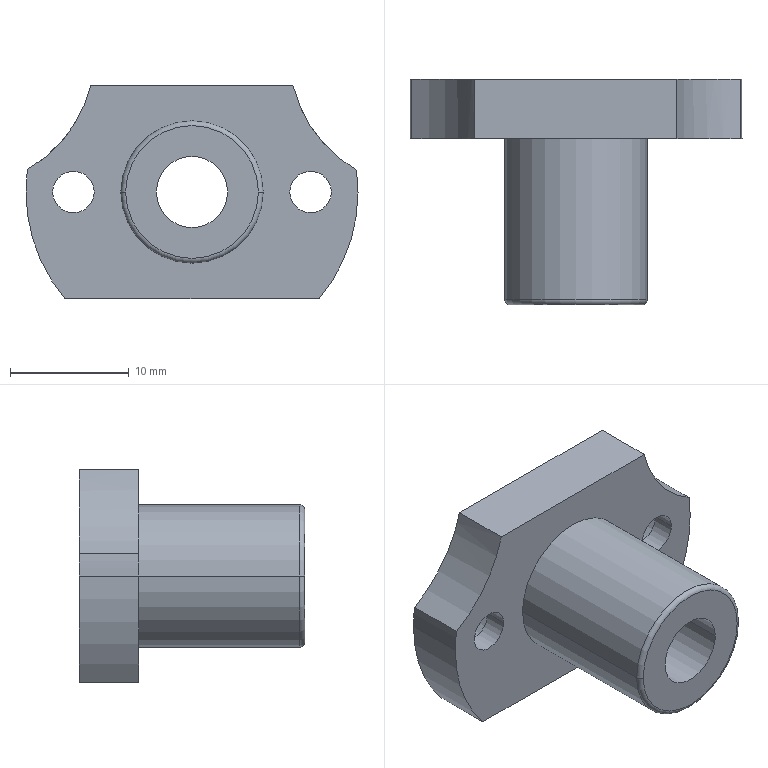Component | SolidWorks | LME21-d6-1 | 1 solid | 26 faces | box 28 x 19 x 18 mm | volume 3005 mm3 | cylinder 17 | plane 7 | torus 2 | commonest cylinder face diameters 6 x6 3.5 x4 28 x3 12 x2 22.6 x2
build123d program:
from build123d import *

# Parameters (mm, degrees)
BOSS_EXTRUDE1_START        = 5
SKETCH2_R                  = 6
BOSS_EXTRUDE1_DEPTH        = 5
FLANGENUTRELIEF_DEPTH      = 26.259
FLANGENUTRELIEF_DEPTH_BACK = 26.259
SKETCH1_R                  = 11.3


with BuildPart() as part:
    # Sketch1_2 → Revolve1 (revolve)
    with BuildSketch(Plane(origin=(0, 0, 0), x_dir=(1, 0, 0), z_dir=(0, 1, 0))):
        with BuildLine():
            Line((-5.6, -19), (-3, -19))
            Line((-3, -19), (-3, 0))
            Line((-3, 0), (-6, 0))
            Line((-6, 0), (-6, -18.6))
            ThreePointArc((-6, -18.6), (-5.883, -18.883), (-5.6, -19))
        make_face()
    revolve(axis=Axis((0, 0, 0), (0, 0, 1)))

    # Sketch2 → Boss-Extrude1 (add)
    with BuildSketch(Plane.XY.offset(BOSS_EXTRUDE1_START)):
        with BuildLine():
            Line((-10.724, -9), (10.724, -9))
            ThreePointArc((10.724, -9), (14, 0), (10.724, 9))
            Line((10.724, 9), (-10.724, 9))
            ThreePointArc((-10.724, 9), (-14, 0), (-10.724, -9))
        make_face()
        with Locations(Location((0, 0, 0), (0, 0, 180))):
            Circle(SKETCH2_R, mode=Mode.SUBTRACT)
    extrude(amount=-BOSS_EXTRUDE1_DEPTH)

    # Sketch3 → Cut-Revolve1 (revolve, cut)
    with BuildSketch(Plane(origin=(0, 0, 0), x_dir=(1, 0, 0), z_dir=(0, 1, 0))):
        Polygon((-10, -5), (-11.75, -5), (-11.75, -3.1), (-13, -3.1), (-13, 0), (-10, 0), align=None)
    revolve(axis=Axis((-10, 0, 0), (0, 0, 1)), mode=Mode.SUBTRACT)

    # Sketch4 → Cut-Revolve2 (revolve, cut)
    with BuildSketch(Plane(origin=(0, 0, 0), x_dir=(1, 0, 0), z_dir=(0, 1, 0))):
        Polygon((10, 0), (13, 0), (13, -3.1), (11.75, -3.1), (11.75, -5), (10, -5), align=None)
    revolve(axis=Axis((10, 0, 5), (0, 0, -1)), mode=Mode.SUBTRACT)

    # Sketch1 → FlangeNutRelief (cut, two sides: drawn at the far end of the back side and taken through both)
    with BuildSketch(Plane.XY.offset(-FLANGENUTRELIEF_DEPTH_BACK)):
        with Locations((19.5, 11.652)):
            Circle(SKETCH1_R)
        with Locations((-19.5, 11.704)):
            Circle(SKETCH1_R)
    extrude(amount=FLANGENUTRELIEF_DEPTH + FLANGENUTRELIEF_DEPTH_BACK, mode=Mode.SUBTRACT)


solid = part.part

# Placed as in the assembly
solid = solid.moved(Location((-57.536, 63.25, 217.788), (90, 0, 0)))
STEP:
#1=COLOUR_RGB('',0.7922,0.8196,0.9333);
#2=FILL_AREA_STYLE_COLOUR('',#1);
#3=FILL_AREA_STYLE('',(#2));
#4=SURFACE_STYLE_FILL_AREA(#3);
#5=SURFACE_SIDE_STYLE('',(#4));
#6=SURFACE_STYLE_USAGE(.BOTH.,#5);
#7=PRESENTATION_STYLE_ASSIGNMENT((#6));
#8=CARTESIAN_POINT('',(-1.94,2.368,8.574));
#9=VERTEX_POINT('',#8);
#10=CARTESIAN_POINT('',(-1.803,2.368,8.574));
#11=VERTEX_POINT('',#10);
#12=CARTESIAN_POINT('',(-1.872,2.368,8.574));
#13=DIRECTION('',(-0.,-1.,0.));
#14=DIRECTION('',(1.,-0.,0.));
#15=AXIS2_PLACEMENT_3D('',#12,#13,#14);
#16=CIRCLE('',#15,0.0689);
#17=EDGE_CURVE('',#9,#11,#16,.T.);
#18=ORIENTED_EDGE('',*,*,#17,.F.);
#19=CARTESIAN_POINT('',(-1.94,2.293,8.574));
#20=VERTEX_POINT('',#19);
#21=CARTESIAN_POINT('',(-1.94,2.293,8.574));
#22=DIRECTION('',(-0.,-1.,0.));
#23=VECTOR('',#22,39.37);
#24=LINE('',#21,#23);
#25=EDGE_CURVE('',#9,#20,#24,.T.);
#26=ORIENTED_EDGE('',*,*,#25,.T.);
#27=CARTESIAN_POINT('',(-1.803,2.293,8.574));
#28=VERTEX_POINT('',#27);
#29=CARTESIAN_POINT('',(-1.872,2.293,8.574));
#30=DIRECTION('',(-0.,-1.,0.));
#31=DIRECTION('',(1.,-0.,0.));
#32=AXIS2_PLACEMENT_3D('',#29,#30,#31);
#33=CIRCLE('',#32,0.0689);
#34=EDGE_CURVE('',#20,#28,#33,.T.);
#35=ORIENTED_EDGE('',*,*,#34,.T.);
#36=CARTESIAN_POINT('',(-1.803,2.293,8.574));
#37=DIRECTION('',(-0.,-1.,0.));
#38=VECTOR('',#37,39.37);
#39=LINE('',#36,#38);
#40=EDGE_CURVE('',#11,#28,#39,.T.);
#41=ORIENTED_EDGE('',*,*,#40,.F.);
#42=EDGE_LOOP('',(#18,#26,#35,#41));
#43=FACE_OUTER_BOUND('',#42,.T.);
#44=CARTESIAN_POINT('',(-1.872,2.293,8.574));
#45=DIRECTION('',(-0.,-1.,0.));
#46=DIRECTION('',(1.,-0.,0.));
#47=AXIS2_PLACEMENT_3D('',#44,#45,#46);
#48=CYLINDRICAL_SURFACE('',#47,0.0689);
#49=ADVANCED_FACE('',(#43),#48,.F.);
#50=CARTESIAN_POINT('',(-1.99,2.49,8.574));
#51=VERTEX_POINT('',#50);
#52=CARTESIAN_POINT('',(-1.753,2.49,8.574));
#53=VERTEX_POINT('',#52);
#54=CARTESIAN_POINT('',(-1.872,2.49,8.574));
#55=DIRECTION('',(-0.,-1.,0.));
#56=DIRECTION('',(1.,-0.,0.));
#57=AXIS2_PLACEMENT_3D('',#54,#55,#56);
#58=CIRCLE('',#57,0.1181);
#59=EDGE_CURVE('',#51,#53,#58,.T.);
#60=ORIENTED_EDGE('',*,*,#59,.F.);
#61=CARTESIAN_POINT('',(-1.99,2.368,8.574));
#62=VERTEX_POINT('',#61);
#63=CARTESIAN_POINT('',(-1.99,2.293,8.574));
#64=DIRECTION('',(-0.,-1.,0.));
#65=VECTOR('',#64,39.37);
#66=LINE('',#63,#65);
#67=EDGE_CURVE('',#51,#62,#66,.T.);
#68=ORIENTED_EDGE('',*,*,#67,.T.);
#69=CARTESIAN_POINT('',(-1.753,2.368,8.574));
#70=VERTEX_POINT('',#69);
#71=CARTESIAN_POINT('',(-1.872,2.368,8.574));
#72=DIRECTION('',(-0.,-1.,0.));
#73=DIRECTION('',(1.,-0.,0.));
#74=AXIS2_PLACEMENT_3D('',#71,#72,#73);
#75=CIRCLE('',#74,0.1181);
#76=EDGE_CURVE('',#62,#70,#75,.T.);
#77=ORIENTED_EDGE('',*,*,#76,.T.);
#78=CARTESIAN_POINT('',(-1.753,2.293,8.574));
#79=DIRECTION('',(-0.,-1.,0.));
#80=VECTOR('',#79,39.37);
#81=LINE('',#78,#80);
#82=EDGE_CURVE('',#53,#70,#81,.T.);
#83=ORIENTED_EDGE('',*,*,#82,.F.);
#84=EDGE_LOOP('',(#60,#68,#77,#83));
#85=FACE_OUTER_BOUND('',#84,.T.);
#86=CARTESIAN_POINT('',(-1.872,2.293,8.574));
#87=DIRECTION('',(-0.,-1.,0.));
#88=DIRECTION('',(1.,-0.,0.));
#89=AXIS2_PLACEMENT_3D('',#86,#87,#88);
#90=CYLINDRICAL_SURFACE('',#89,0.1181);
#91=ADVANCED_FACE('',(#85),#90,.F.);
#92=CARTESIAN_POINT('',(-2.541,2.368,8.574));
#93=VERTEX_POINT('',#92);
#94=CARTESIAN_POINT('',(-2.777,2.368,8.574));
#95=VERTEX_POINT('',#94);
#96=CARTESIAN_POINT('',(-2.659,2.368,8.574));
#97=DIRECTION('',(0.,1.,-0.));
#98=DIRECTION('',(-1.,0.,-0.));
#99=AXIS2_PLACEMENT_3D('',#96,#97,#98);
#100=CIRCLE('',#99,0.1181);
#101=EDGE_CURVE('',#93,#95,#100,.T.);
#102=ORIENTED_EDGE('',*,*,#101,.F.);
#103=CARTESIAN_POINT('',(-2.541,2.49,8.574));
#104=VERTEX_POINT('',#103);
#105=CARTESIAN_POINT('',(-2.541,2.49,8.574));
#106=DIRECTION('',(0.,1.,-0.));
#107=VECTOR('',#106,39.37);
#108=LINE('',#105,#107);
#109=EDGE_CURVE('',#93,#104,#108,.T.);
#110=ORIENTED_EDGE('',*,*,#109,.T.);
#111=CARTESIAN_POINT('',(-2.777,2.49,8.574));
#112=VERTEX_POINT('',#111);
#113=CARTESIAN_POINT('',(-2.659,2.49,8.574));
#114=DIRECTION('',(0.,1.,-0.));
#115=DIRECTION('',(-1.,0.,-0.));
#116=AXIS2_PLACEMENT_3D('',#113,#114,#115);
#117=CIRCLE('',#116,0.1181);
#118=EDGE_CURVE('',#104,#112,#117,.T.);
#119=ORIENTED_EDGE('',*,*,#118,.T.);
#120=CARTESIAN_POINT('',(-2.777,2.49,8.574));
#121=DIRECTION('',(0.,1.,-0.));
#122=VECTOR('',#121,39.37);
#123=LINE('',#120,#122);
#124=EDGE_CURVE('',#95,#112,#123,.T.);
#125=ORIENTED_EDGE('',*,*,#124,.F.);
#126=EDGE_LOOP('',(#102,#110,#119,#125));
#127=FACE_OUTER_BOUND('',#126,.T.);
#128=CARTESIAN_POINT('',(-2.659,2.49,8.574));
#129=DIRECTION('',(0.,1.,-0.));
#130=DIRECTION('',(-1.,0.,-0.));
#131=AXIS2_PLACEMENT_3D('',#128,#129,#130);
#132=CYLINDRICAL_SURFACE('',#131,0.1181);
#133=ADVANCED_FACE('',(#127),#132,.F.);
#134=CARTESIAN_POINT('',(-2.59,2.293,8.574));
#135=VERTEX_POINT('',#134);
#136=CARTESIAN_POINT('',(-2.728,2.293,8.574));
#137=VERTEX_POINT('',#136);
#138=CARTESIAN_POINT('',(-2.659,2.293,8.574));
#139=DIRECTION('',(0.,1.,-0.));
#140=DIRECTION('',(-1.,0.,0.));
#141=AXIS2_PLACEMENT_3D('',#138,#139,#140);
#142=CIRCLE('',#141,0.0689);
#143=EDGE_CURVE('',#135,#137,#142,.T.);
#144=ORIENTED_EDGE('',*,*,#143,.F.);
#145=CARTESIAN_POINT('',(-2.59,2.368,8.574));
#146=VERTEX_POINT('',#145);
#147=CARTESIAN_POINT('',(-2.59,2.49,8.574));
#148=DIRECTION('',(0.,1.,-0.));
#149=VECTOR('',#148,39.37);
#150=LINE('',#147,#149);
#151=EDGE_CURVE('',#135,#146,#150,.T.);
#152=ORIENTED_EDGE('',*,*,#151,.T.);
#153=CARTESIAN_POINT('',(-2.728,2.368,8.574));
#154=VERTEX_POINT('',#153);
#155=CARTESIAN_POINT('',(-2.659,2.368,8.574));
#156=DIRECTION('',(0.,1.,-0.));
#157=DIRECTION('',(-1.,0.,0.));
#158=AXIS2_PLACEMENT_3D('',#155,#156,#157);
#159=CIRCLE('',#158,0.0689);
#160=EDGE_CURVE('',#146,#154,#159,.T.);
#161=ORIENTED_EDGE('',*,*,#160,.T.);
#162=CARTESIAN_POINT('',(-2.728,2.49,8.574));
#163=DIRECTION('',(0.,1.,-0.));
#164=VECTOR('',#163,39.37);
#165=LINE('',#162,#164);
#166=EDGE_CURVE('',#137,#154,#165,.T.);
#167=ORIENTED_EDGE('',*,*,#166,.F.);
#168=EDGE_LOOP('',(#144,#152,#161,#167));
#169=FACE_OUTER_BOUND('',#168,.T.);
#170=CARTESIAN_POINT('',(-2.659,2.49,8.574));
#171=DIRECTION('',(0.,1.,-0.));
#172=DIRECTION('',(-1.,0.,0.));
#173=AXIS2_PLACEMENT_3D('',#170,#171,#172);
#174=CYLINDRICAL_SURFACE('',#173,0.0689);
#175=ADVANCED_FACE('',(#169),#174,.F.);
#176=CARTESIAN_POINT('',(-2.816,2.293,8.574));
#177=VERTEX_POINT('',#176);
#178=CARTESIAN_POINT('',(-2.687,2.293,8.22));
#179=VERTEX_POINT('',#178);
#180=CARTESIAN_POINT('',(-2.265,2.293,8.574));
#181=DIRECTION('',(-0.,-1.,0.));
#182=DIRECTION('',(1.,-0.,0.));
#183=AXIS2_PLACEMENT_3D('',#180,#181,#182);
#184=CIRCLE('',#183,0.5512);
#185=EDGE_CURVE('',#177,#179,#184,.T.);
#186=ORIENTED_EDGE('',*,*,#185,.F.);
#187=CARTESIAN_POINT('',(-2.816,2.49,8.574));
#188=VERTEX_POINT('',#187);
#189=CARTESIAN_POINT('',(-2.816,2.293,8.574));
#190=DIRECTION('',(0.,1.,-0.));
#191=VECTOR('',#190,39.37);
#192=LINE('',#189,#191);
#193=EDGE_CURVE('',#177,#188,#192,.T.);
#194=ORIENTED_EDGE('',*,*,#193,.T.);
#195=CARTESIAN_POINT('',(-2.687,2.49,8.22));
#196=VERTEX_POINT('',#195);
#197=CARTESIAN_POINT('',(-2.265,2.49,8.574));
#198=DIRECTION('',(-0.,-1.,0.));
#199=DIRECTION('',(1.,-0.,0.));
#200=AXIS2_PLACEMENT_3D('',#197,#198,#199);
#201=CIRCLE('',#200,0.5512);
#202=EDGE_CURVE('',#188,#196,#201,.T.);
#203=ORIENTED_EDGE('',*,*,#202,.T.);
#204=CARTESIAN_POINT('',(-2.687,2.293,8.22));
#205=DIRECTION('',(0.,1.,-0.));
#206=VECTOR('',#205,39.37);
#207=LINE('',#204,#206);
#208=EDGE_CURVE('',#179,#196,#207,.T.);
#209=ORIENTED_EDGE('',*,*,#208,.F.);
#210=EDGE_LOOP('',(#186,#194,#203,#209));
#211=FACE_OUTER_BOUND('',#210,.T.);
#212=CARTESIAN_POINT('',(-2.265,2.293,8.574));
#213=DIRECTION('',(0.,1.,-0.));
#214=DIRECTION('',(-1.,0.,-0.));
#215=AXIS2_PLACEMENT_3D('',#212,#213,#214);
#216=CYLINDRICAL_SURFACE('',#215,0.5512);
#217=ADVANCED_FACE('',(#211),#216,.T.);
#218=CARTESIAN_POINT('',(-2.501,1.758,8.574));
#219=VERTEX_POINT('',#218);
#220=CARTESIAN_POINT('',(-2.029,1.758,8.574));
#221=VERTEX_POINT('',#220);
#222=CARTESIAN_POINT('',(-2.265,1.758,8.574));
#223=DIRECTION('',(0.,1.,-0.));
#224=DIRECTION('',(-1.,0.,-0.));
#225=AXIS2_PLACEMENT_3D('',#222,#223,#224);
#226=CIRCLE('',#225,0.2362);
#227=EDGE_CURVE('',#219,#221,#226,.T.);
#228=ORIENTED_EDGE('',*,*,#227,.T.);
#229=CARTESIAN_POINT('',(-2.029,2.293,8.574));
#230=VERTEX_POINT('',#229);
#231=CARTESIAN_POINT('',(-2.029,2.49,8.574));
#232=DIRECTION('',(0.,1.,-0.));
#233=VECTOR('',#232,39.37);
#234=LINE('',#231,#233);
#235=EDGE_CURVE('',#221,#230,#234,.T.);
#236=ORIENTED_EDGE('',*,*,#235,.T.);
#237=CARTESIAN_POINT('',(-2.501,2.293,8.574));
#238=VERTEX_POINT('',#237);
#239=CARTESIAN_POINT('',(-2.265,2.293,8.574));
#240=DIRECTION('',(0.,1.,-0.));
#241=DIRECTION('',(1.,-0.,0.));
#242=AXIS2_PLACEMENT_3D('',#239,#240,#241);
#243=CIRCLE('',#242,0.2362);
#244=EDGE_CURVE('',#238,#230,#243,.T.);
#245=ORIENTED_EDGE('',*,*,#244,.F.);
#246=CARTESIAN_POINT('',(-2.501,2.49,8.574));
#247=DIRECTION('',(0.,1.,-0.));
#248=VECTOR('',#247,39.37);
#249=LINE('',#246,#248);
#250=EDGE_CURVE('',#219,#238,#249,.T.);
#251=ORIENTED_EDGE('',*,*,#250,.F.);
#252=EDGE_LOOP('',(#228,#236,#245,#251));
#253=FACE_OUTER_BOUND('',#252,.T.);
#254=CARTESIAN_POINT('',(-2.265,2.49,8.574));
#255=DIRECTION('',(0.,1.,-0.));
#256=DIRECTION('',(-1.,0.,-0.));
#257=AXIS2_PLACEMENT_3D('',#254,#255,#256);
#258=CYLINDRICAL_SURFACE('',#257,0.2362);
#259=ADVANCED_FACE('',(#253),#258,.T.);
#260=CARTESIAN_POINT('',(-2.147,1.742,8.574));
#261=VERTEX_POINT('',#260);
#262=CARTESIAN_POINT('',(-2.383,1.742,8.574));
#263=VERTEX_POINT('',#262);
#264=CARTESIAN_POINT('',(-2.265,1.742,8.574));
#265=DIRECTION('',(0.,1.,-0.));
#266=DIRECTION('',(-1.,0.,-0.));
#267=AXIS2_PLACEMENT_3D('',#264,#265,#266);
#268=CIRCLE('',#267,0.1181);
#269=EDGE_CURVE('',#261,#263,#268,.T.);
#270=ORIENTED_EDGE('',*,*,#269,.F.);
#271=CARTESIAN_POINT('',(-2.147,2.49,8.574));
#272=VERTEX_POINT('',#271);
#273=CARTESIAN_POINT('',(-2.147,2.49,8.574));
#274=DIRECTION('',(0.,1.,-0.));
#275=VECTOR('',#274,39.37);
#276=LINE('',#273,#275);
#277=EDGE_CURVE('',#261,#272,#276,.T.);
#278=ORIENTED_EDGE('',*,*,#277,.T.);
#279=CARTESIAN_POINT('',(-2.383,2.49,8.574));
#280=VERTEX_POINT('',#279);
#281=CARTESIAN_POINT('',(-2.265,2.49,8.574));
#282=DIRECTION('',(0.,1.,-0.));
#283=DIRECTION('',(-1.,0.,-0.));
#284=AXIS2_PLACEMENT_3D('',#281,#282,#283);
#285=CIRCLE('',#284,0.1181);
#286=EDGE_CURVE('',#272,#280,#285,.T.);
#287=ORIENTED_EDGE('',*,*,#286,.T.);
#288=CARTESIAN_POINT('',(-2.383,2.49,8.574));
#289=DIRECTION('',(0.,1.,-0.));
#290=VECTOR('',#289,39.37);
#291=LINE('',#288,#290);
#292=EDGE_CURVE('',#263,#280,#291,.T.);
#293=ORIENTED_EDGE('',*,*,#292,.F.);
#294=EDGE_LOOP('',(#270,#278,#287,#293));
#295=FACE_OUTER_BOUND('',#294,.T.);
#296=CARTESIAN_POINT('',(-2.265,2.49,8.574));
#297=DIRECTION('',(0.,1.,-0.));
#298=DIRECTION('',(-1.,0.,-0.));
#299=AXIS2_PLACEMENT_3D('',#296,#297,#298);
#300=CYLINDRICAL_SURFACE('',#299,0.1181);
#301=ADVANCED_FACE('',(#295),#300,.F.);
#302=CARTESIAN_POINT('',(-2.486,1.742,8.574));
#303=VERTEX_POINT('',#302);
#304=CARTESIAN_POINT('',(-2.045,1.742,8.574));
#305=VERTEX_POINT('',#304);
#306=CARTESIAN_POINT('',(-2.265,1.742,8.574));
#307=DIRECTION('',(0.,1.,-0.));
#308=DIRECTION('',(-1.,0.,-0.));
#309=AXIS2_PLACEMENT_3D('',#306,#307,#308);
#310=CIRCLE('',#309,0.2205);
#311=EDGE_CURVE('',#303,#305,#310,.T.);
#312=ORIENTED_EDGE('',*,*,#311,.T.);
#313=CARTESIAN_POINT('',(-2.045,1.758,8.574));
#314=DIRECTION('',(-0.,0.,1.));
#315=DIRECTION('',(1.,0.,0.));
#316=AXIS2_PLACEMENT_3D('',#313,#314,#315);
#317=CIRCLE('',#316,0.01575);
#318=EDGE_CURVE('',#305,#221,#317,.T.);
#319=ORIENTED_EDGE('',*,*,#318,.T.);
#320=ORIENTED_EDGE('',*,*,#227,.F.);
#321=CARTESIAN_POINT('',(-2.486,1.758,8.574));
#322=DIRECTION('',(0.,-0.,-1.));
#323=DIRECTION('',(-1.,0.,0.));
#324=AXIS2_PLACEMENT_3D('',#321,#322,#323);
#325=CIRCLE('',#324,0.01575);
#326=EDGE_CURVE('',#303,#219,#325,.T.);
#327=ORIENTED_EDGE('',*,*,#326,.F.);
#328=EDGE_LOOP('',(#312,#319,#320,#327));
#329=FACE_OUTER_BOUND('',#328,.T.);
#330=CARTESIAN_POINT('',(-2.265,1.758,8.574));
#331=DIRECTION('',(0.,1.,-0.));
#332=DIRECTION('',(-1.,0.,-0.));
#333=AXIS2_PLACEMENT_3D('',#330,#331,#332);
#334=TOROIDAL_SURFACE('',#333,0.2205,0.01575);
#335=ADVANCED_FACE('',(#329),#334,.T.);
#336=CARTESIAN_POINT('',(-1.872,2.49,8.574));
#337=DIRECTION('',(-0.,-1.,0.));
#338=DIRECTION('',(1.,-0.,0.));
#339=AXIS2_PLACEMENT_3D('',#336,#337,#338);
#340=CIRCLE('',#339,0.1181);
#341=EDGE_CURVE('',#53,#51,#340,.T.);
#342=ORIENTED_EDGE('',*,*,#341,.T.);
#343=ORIENTED_EDGE('',*,*,#59,.T.);
#344=EDGE_LOOP('',(#342,#343));
#345=FACE_BOUND('',#344,.T.);
#346=CARTESIAN_POINT('',(-2.659,2.49,8.574));
#347=DIRECTION('',(0.,1.,-0.));
#348=DIRECTION('',(-1.,0.,-0.));
#349=AXIS2_PLACEMENT_3D('',#346,#347,#348);
#350=CIRCLE('',#349,0.1181);
#351=EDGE_CURVE('',#112,#104,#350,.T.);
#352=ORIENTED_EDGE('',*,*,#351,.F.);
#353=ORIENTED_EDGE('',*,*,#118,.F.);
#354=EDGE_LOOP('',(#352,#353));
#355=FACE_BOUND('',#354,.T.);
#356=CARTESIAN_POINT('',(-2.265,2.49,8.574));
#357=DIRECTION('',(0.,1.,-0.));
#358=DIRECTION('',(-1.,0.,-0.));
#359=AXIS2_PLACEMENT_3D('',#356,#357,#358);
#360=CIRCLE('',#359,0.1181);
#361=EDGE_CURVE('',#280,#272,#360,.T.);
#362=ORIENTED_EDGE('',*,*,#361,.F.);
#363=ORIENTED_EDGE('',*,*,#286,.F.);
#364=EDGE_LOOP('',(#362,#363));
#365=FACE_BOUND('',#364,.T.);
#366=CARTESIAN_POINT('',(-1.93,2.49,8.929));
#367=VERTEX_POINT('',#366);
#368=CARTESIAN_POINT('',(-2.601,2.49,8.929));
#369=VERTEX_POINT('',#368);
#370=CARTESIAN_POINT('',(-1.843,2.49,8.929));
#371=DIRECTION('',(-1.,0.,-0.));
#372=VECTOR('',#371,39.37);
#373=LINE('',#370,#372);
#374=EDGE_CURVE('',#367,#369,#373,.T.);
#375=ORIENTED_EDGE('',*,*,#374,.F.);
#376=CARTESIAN_POINT('',(-1.719,2.49,8.647));
#377=VERTEX_POINT('',#376);
#378=CARTESIAN_POINT('',(-1.93,2.49,8.929));
#379=CARTESIAN_POINT('',(-1.926,2.49,8.914));
#380=CARTESIAN_POINT('',(-1.922,2.49,8.9));
#381=CARTESIAN_POINT('',(-1.912,2.49,8.871));
#382=CARTESIAN_POINT('',(-1.906,2.49,8.857));
#383=CARTESIAN_POINT('',(-1.887,2.49,8.816));
#384=CARTESIAN_POINT('',(-1.864,2.49,8.777));
#385=CARTESIAN_POINT('',(-1.835,2.49,8.743));
#386=CARTESIAN_POINT('',(-1.814,2.49,8.72));
#387=CARTESIAN_POINT('',(-1.803,2.49,8.71));
#388=CARTESIAN_POINT('',(-1.769,2.49,8.679));
#389=CARTESIAN_POINT('',(-1.745,2.49,8.662));
#390=CARTESIAN_POINT('',(-1.719,2.49,8.647));
#391=B_SPLINE_CURVE_WITH_KNOTS('',3,(#378,#379,#380,#381,#382,#383,#384,#385,#386,#387,#388,#389,#390),.UNSPECIFIED.,.F.,.F.,(4,2,2,1,2,2,4),(0.5377,0.5539,0.5701,0.6025,0.6186,0.6348,0.6672),.UNSPECIFIED.);
#392=EDGE_CURVE('',#367,#377,#391,.T.);
#393=ORIENTED_EDGE('',*,*,#392,.T.);
#394=CARTESIAN_POINT('',(-1.843,2.49,8.22));
#395=VERTEX_POINT('',#394);
#396=CARTESIAN_POINT('',(-2.265,2.49,8.574));
#397=DIRECTION('',(-0.,-1.,0.));
#398=DIRECTION('',(1.,-0.,0.));
#399=AXIS2_PLACEMENT_3D('',#396,#397,#398);
#400=CIRCLE('',#399,0.5512);
#401=EDGE_CURVE('',#395,#377,#400,.T.);
#402=ORIENTED_EDGE('',*,*,#401,.F.);
#403=CARTESIAN_POINT('',(-2.687,2.49,8.22));
#404=DIRECTION('',(1.,-0.,0.));
#405=VECTOR('',#404,39.37);
#406=LINE('',#403,#405);
#407=EDGE_CURVE('',#196,#395,#406,.T.);
#408=ORIENTED_EDGE('',*,*,#407,.F.);
#409=ORIENTED_EDGE('',*,*,#202,.F.);
#410=CARTESIAN_POINT('',(-2.811,2.49,8.649));
#411=VERTEX_POINT('',#410);
#412=CARTESIAN_POINT('',(-2.265,2.49,8.574));
#413=DIRECTION('',(-0.,-1.,0.));
#414=DIRECTION('',(1.,-0.,0.));
#415=AXIS2_PLACEMENT_3D('',#412,#413,#414);
#416=CIRCLE('',#415,0.5512);
#417=EDGE_CURVE('',#411,#188,#416,.T.);
#418=ORIENTED_EDGE('',*,*,#417,.F.);
#419=CARTESIAN_POINT('',(-2.811,2.49,8.649));
#420=CARTESIAN_POINT('',(-2.785,2.49,8.664));
#421=CARTESIAN_POINT('',(-2.761,2.49,8.682));
#422=CARTESIAN_POINT('',(-2.727,2.49,8.711));
#423=CARTESIAN_POINT('',(-2.717,2.49,8.722));
#424=CARTESIAN_POINT('',(-2.696,2.49,8.744));
#425=CARTESIAN_POINT('',(-2.667,2.49,8.779));
#426=CARTESIAN_POINT('',(-2.644,2.49,8.817));
#427=CARTESIAN_POINT('',(-2.625,2.49,8.858));
#428=CARTESIAN_POINT('',(-2.619,2.49,8.872));
#429=CARTESIAN_POINT('',(-2.609,2.49,8.9));
#430=CARTESIAN_POINT('',(-2.604,2.49,8.914));
#431=CARTESIAN_POINT('',(-2.601,2.49,8.929));
#432=B_SPLINE_CURVE_WITH_KNOTS('',3,(#419,#420,#421,#422,#423,#424,#425,#426,#427,#428,#429,#430,#431),.UNSPECIFIED.,.F.,.F.,(4,2,2,1,2,2,4),(0.8329,0.8651,0.8812,0.8972,0.9294,0.9454,0.9615),.UNSPECIFIED.);
#433=EDGE_CURVE('',#411,#369,#432,.T.);
#434=ORIENTED_EDGE('',*,*,#433,.T.);
#435=EDGE_LOOP('',(#375,#393,#402,#408,#409,#418,#434));
#436=FACE_OUTER_BOUND('',#435,.T.);
#437=CARTESIAN_POINT('',(-2.383,2.49,8.574));
#438=DIRECTION('',(0.,1.,-0.));
#439=DIRECTION('',(-1.,0.,-0.));
#440=AXIS2_PLACEMENT_3D('',#437,#438,#439);
#441=PLANE('',#440);
#442=ADVANCED_FACE('',(#345,#355,#365,#436),#441,.T.);
#443=ORIENTED_EDGE('',*,*,#318,.F.);
#444=CARTESIAN_POINT('',(-2.265,1.742,8.574));
#445=DIRECTION('',(0.,1.,-0.));
#446=DIRECTION('',(-1.,0.,-0.));
#447=AXIS2_PLACEMENT_3D('',#444,#445,#446);
#448=CIRCLE('',#447,0.2205);
#449=EDGE_CURVE('',#305,#303,#448,.T.);
#450=ORIENTED_EDGE('',*,*,#449,.T.);
#451=ORIENTED_EDGE('',*,*,#326,.T.);
#452=CARTESIAN_POINT('',(-2.265,1.758,8.574));
#453=DIRECTION('',(0.,1.,-0.));
#454=DIRECTION('',(-1.,0.,-0.));
#455=AXIS2_PLACEMENT_3D('',#452,#453,#454);
#456=CIRCLE('',#455,0.2362);
#457=EDGE_CURVE('',#221,#219,#456,.T.);
#458=ORIENTED_EDGE('',*,*,#457,.F.);
#459=EDGE_LOOP('',(#443,#450,#451,#458));
#460=FACE_OUTER_BOUND('',#459,.T.);
#461=CARTESIAN_POINT('',(-2.265,1.758,8.574));
#462=DIRECTION('',(0.,1.,-0.));
#463=DIRECTION('',(-1.,0.,-0.));
#464=AXIS2_PLACEMENT_3D('',#461,#462,#463);
#465=TOROIDAL_SURFACE('',#464,0.2205,0.01575);
#466=ADVANCED_FACE('',(#460),#465,.T.);
#467=CARTESIAN_POINT('',(-2.265,1.742,8.574));
#468=DIRECTION('',(0.,1.,-0.));
#469=DIRECTION('',(-1.,0.,-0.));
#470=AXIS2_PLACEMENT_3D('',#467,#468,#469);
#471=CIRCLE('',#470,0.1181);
#472=EDGE_CURVE('',#263,#261,#471,.T.);
#473=ORIENTED_EDGE('',*,*,#472,.T.);
#474=ORIENTED_EDGE('',*,*,#269,.T.);
#475=EDGE_LOOP('',(#473,#474));
#476=FACE_BOUND('',#475,.T.);
#477=ORIENTED_EDGE('',*,*,#311,.F.);
#478=ORIENTED_EDGE('',*,*,#449,.F.);
#479=EDGE_LOOP('',(#477,#478));
#480=FACE_OUTER_BOUND('',#479,.T.);
#481=CARTESIAN_POINT('',(-2.486,1.742,8.574));
#482=DIRECTION('',(-0.,-1.,0.));
#483=DIRECTION('',(1.,-0.,0.));
#484=AXIS2_PLACEMENT_3D('',#481,#482,#483);
#485=PLANE('',#484);
#486=ADVANCED_FACE('',(#476,#480),#485,.T.);
#487=ORIENTED_EDGE('',*,*,#277,.F.);
#488=ORIENTED_EDGE('',*,*,#472,.F.);
#489=ORIENTED_EDGE('',*,*,#292,.T.);
#490=ORIENTED_EDGE('',*,*,#361,.T.);
#491=EDGE_LOOP('',(#487,#488,#489,#490));
#492=FACE_OUTER_BOUND('',#491,.T.);
#493=CARTESIAN_POINT('',(-2.265,2.49,8.574));
#494=DIRECTION('',(0.,1.,-0.));
#495=DIRECTION('',(-1.,0.,-0.));
#496=AXIS2_PLACEMENT_3D('',#493,#494,#495);
#497=CYLINDRICAL_SURFACE('',#496,0.1181);
#498=ADVANCED_FACE('',(#492),#497,.F.);
#499=ORIENTED_EDGE('',*,*,#235,.F.);
#500=ORIENTED_EDGE('',*,*,#457,.T.);
#501=ORIENTED_EDGE('',*,*,#250,.T.);
#502=CARTESIAN_POINT('',(-2.265,2.293,8.574));
#503=DIRECTION('',(0.,1.,-0.));
#504=DIRECTION('',(1.,-0.,0.));
#505=AXIS2_PLACEMENT_3D('',#502,#503,#504);
#506=CIRCLE('',#505,0.2362);
#507=EDGE_CURVE('',#230,#238,#506,.T.);
#508=ORIENTED_EDGE('',*,*,#507,.F.);
#509=EDGE_LOOP('',(#499,#500,#501,#508));
#510=FACE_OUTER_BOUND('',#509,.T.);
#511=CARTESIAN_POINT('',(-2.265,2.49,8.574));
#512=DIRECTION('',(0.,1.,-0.));
#513=DIRECTION('',(-1.,0.,-0.));
#514=AXIS2_PLACEMENT_3D('',#511,#512,#513);
#515=CYLINDRICAL_SURFACE('',#514,0.2362);
#516=ADVANCED_FACE('',(#510),#515,.T.);
#517=CARTESIAN_POINT('',(-1.93,2.293,8.929));
#518=VERTEX_POINT('',#517);
#519=CARTESIAN_POINT('',(-1.719,2.293,8.647));
#520=VERTEX_POINT('',#519);
#521=CARTESIAN_POINT('',(-1.497,2.293,9.033));
#522=DIRECTION('',(-0.,-1.,0.));
#523=DIRECTION('',(1.,-0.,0.));
#524=AXIS2_PLACEMENT_3D('',#521,#522,#523);
#525=CIRCLE('',#524,0.4449);
#526=EDGE_CURVE('',#518,#520,#525,.T.);
#527=ORIENTED_EDGE('',*,*,#526,.F.);
#528=CARTESIAN_POINT('',(-2.601,2.293,8.929));
#529=VERTEX_POINT('',#528);
#530=CARTESIAN_POINT('',(-1.843,2.293,8.929));
#531=DIRECTION('',(-1.,0.,-0.));
#532=VECTOR('',#531,39.37);
#533=LINE('',#530,#532);
#534=EDGE_CURVE('',#518,#529,#533,.T.);
#535=ORIENTED_EDGE('',*,*,#534,.T.);
#536=CARTESIAN_POINT('',(-2.811,2.293,8.649));
#537=VERTEX_POINT('',#536);
#538=CARTESIAN_POINT('',(-3.033,2.293,9.035));
#539=DIRECTION('',(-0.,-1.,0.));
#540=DIRECTION('',(1.,-0.,0.));
#541=AXIS2_PLACEMENT_3D('',#538,#539,#540);
#542=CIRCLE('',#541,0.4449);
#543=EDGE_CURVE('',#537,#529,#542,.T.);
#544=ORIENTED_EDGE('',*,*,#543,.F.);
#545=CARTESIAN_POINT('',(-2.265,2.293,8.574));
#546=DIRECTION('',(-0.,-1.,0.));
#547=DIRECTION('',(1.,-0.,0.));
#548=AXIS2_PLACEMENT_3D('',#545,#546,#547);
#549=CIRCLE('',#548,0.5512);
#550=EDGE_CURVE('',#537,#177,#549,.T.);
#551=ORIENTED_EDGE('',*,*,#550,.T.);
#552=ORIENTED_EDGE('',*,*,#185,.T.);
#553=CARTESIAN_POINT('',(-1.843,2.293,8.22));
#554=VERTEX_POINT('',#553);
#555=CARTESIAN_POINT('',(-2.687,2.293,8.22));
#556=DIRECTION('',(1.,-0.,0.));
#557=VECTOR('',#556,39.37);
#558=LINE('',#555,#557);
#559=EDGE_CURVE('',#179,#554,#558,.T.);
#560=ORIENTED_EDGE('',*,*,#559,.T.);
#561=CARTESIAN_POINT('',(-2.265,2.293,8.574));
#562=DIRECTION('',(-0.,-1.,0.));
#563=DIRECTION('',(1.,-0.,0.));
#564=AXIS2_PLACEMENT_3D('',#561,#562,#563);
#565=CIRCLE('',#564,0.5512);
#566=EDGE_CURVE('',#554,#520,#565,.T.);
#567=ORIENTED_EDGE('',*,*,#566,.T.);
#568=EDGE_LOOP('',(#527,#535,#544,#551,#552,#560,#567));
#569=FACE_OUTER_BOUND('',#568,.T.);
#570=CARTESIAN_POINT('',(-1.872,2.293,8.574));
#571=DIRECTION('',(-0.,-1.,0.));
#572=DIRECTION('',(1.,-0.,0.));
#573=AXIS2_PLACEMENT_3D('',#570,#571,#572);
#574=CIRCLE('',#573,0.0689);
#575=EDGE_CURVE('',#28,#20,#574,.T.);
#576=ORIENTED_EDGE('',*,*,#575,.F.);
#577=ORIENTED_EDGE('',*,*,#34,.F.);
#578=EDGE_LOOP('',(#576,#577));
#579=FACE_BOUND('',#578,.T.);
#580=CARTESIAN_POINT('',(-2.659,2.293,8.574));
#581=DIRECTION('',(0.,1.,-0.));
#582=DIRECTION('',(-1.,0.,0.));
#583=AXIS2_PLACEMENT_3D('',#580,#581,#582);
#584=CIRCLE('',#583,0.0689);
#585=EDGE_CURVE('',#137,#135,#584,.T.);
#586=ORIENTED_EDGE('',*,*,#585,.T.);
#587=ORIENTED_EDGE('',*,*,#143,.T.);
#588=EDGE_LOOP('',(#586,#587));
#589=FACE_BOUND('',#588,.T.);
#590=ORIENTED_EDGE('',*,*,#244,.T.);
#591=ORIENTED_EDGE('',*,*,#507,.T.);
#592=EDGE_LOOP('',(#590,#591));
#593=FACE_BOUND('',#592,.T.);
#594=CARTESIAN_POINT('',(-2.265,2.293,8.574));
#595=DIRECTION('',(-0.,-1.,0.));
#596=DIRECTION('',(1.,-0.,0.));
#597=AXIS2_PLACEMENT_3D('',#594,#595,#596);
#598=PLANE('',#597);
#599=ADVANCED_FACE('',(#569,#579,#589,#593),#598,.T.);
#600=ORIENTED_EDGE('',*,*,#193,.F.);
#601=ORIENTED_EDGE('',*,*,#550,.F.);
#602=CARTESIAN_POINT('',(-2.811,2.116,8.649));
#603=DIRECTION('',(0.,1.,-0.));
#604=VECTOR('',#603,39.37);
#605=LINE('',#602,#604);
#606=EDGE_CURVE('',#537,#411,#605,.T.);
#607=ORIENTED_EDGE('',*,*,#606,.T.);
#608=ORIENTED_EDGE('',*,*,#417,.T.);
#609=EDGE_LOOP('',(#600,#601,#607,#608));
#610=FACE_OUTER_BOUND('',#609,.T.);
#611=CARTESIAN_POINT('',(-2.265,2.293,8.574));
#612=DIRECTION('',(0.,1.,-0.));
#613=DIRECTION('',(-1.,0.,-0.));
#614=AXIS2_PLACEMENT_3D('',#611,#612,#613);
#615=CYLINDRICAL_SURFACE('',#614,0.5512);
#616=ADVANCED_FACE('',(#610),#615,.T.);
#617=ORIENTED_EDGE('',*,*,#407,.T.);
#618=CARTESIAN_POINT('',(-1.843,2.293,8.22));
#619=DIRECTION('',(0.,1.,-0.));
#620=VECTOR('',#619,39.37);
#621=LINE('',#618,#620);
#622=EDGE_CURVE('',#554,#395,#621,.T.);
#623=ORIENTED_EDGE('',*,*,#622,.F.);
#624=ORIENTED_EDGE('',*,*,#559,.F.);
#625=ORIENTED_EDGE('',*,*,#208,.T.);
#626=EDGE_LOOP('',(#617,#623,#624,#625));
#627=FACE_OUTER_BOUND('',#626,.T.);
#628=CARTESIAN_POINT('',(-2.687,2.293,8.22));
#629=DIRECTION('',(-0.,0.,1.));
#630=DIRECTION('',(-0.,-1.,0.));
#631=AXIS2_PLACEMENT_3D('',#628,#629,#630);
#632=PLANE('',#631);
#633=ADVANCED_FACE('',(#627),#632,.F.);
#634=ORIENTED_EDGE('',*,*,#401,.T.);
#635=CARTESIAN_POINT('',(-1.719,2.116,8.647));
#636=DIRECTION('',(-0.,-1.,0.));
#637=VECTOR('',#636,39.37);
#638=LINE('',#635,#637);
#639=EDGE_CURVE('',#377,#520,#638,.T.);
#640=ORIENTED_EDGE('',*,*,#639,.T.);
#641=ORIENTED_EDGE('',*,*,#566,.F.);
#642=ORIENTED_EDGE('',*,*,#622,.T.);
#643=EDGE_LOOP('',(#634,#640,#641,#642));
#644=FACE_OUTER_BOUND('',#643,.T.);
#645=CARTESIAN_POINT('',(-2.265,2.293,8.574));
#646=DIRECTION('',(0.,1.,-0.));
#647=DIRECTION('',(-1.,0.,-0.));
#648=AXIS2_PLACEMENT_3D('',#645,#646,#647);
#649=CYLINDRICAL_SURFACE('',#648,0.5512);
#650=ADVANCED_FACE('',(#644),#649,.T.);
#651=ORIENTED_EDGE('',*,*,#534,.F.);
#652=CARTESIAN_POINT('',(-1.93,2.49,8.929));
#653=DIRECTION('',(0.,1.,-0.));
#654=VECTOR('',#653,39.37);
#655=LINE('',#652,#654);
#656=EDGE_CURVE('',#518,#367,#655,.T.);
#657=ORIENTED_EDGE('',*,*,#656,.T.);
#658=ORIENTED_EDGE('',*,*,#374,.T.);
#659=CARTESIAN_POINT('',(-2.601,2.49,8.929));
#660=DIRECTION('',(-0.,-1.,0.));
#661=VECTOR('',#660,39.37);
#662=LINE('',#659,#661);
#663=EDGE_CURVE('',#369,#529,#662,.T.);
#664=ORIENTED_EDGE('',*,*,#663,.T.);
#665=EDGE_LOOP('',(#651,#657,#658,#664));
#666=FACE_OUTER_BOUND('',#665,.T.);
#667=CARTESIAN_POINT('',(-1.843,2.293,8.929));
#668=DIRECTION('',(0.,-0.,-1.));
#669=DIRECTION('',(0.,1.,-0.));
#670=AXIS2_PLACEMENT_3D('',#667,#668,#669);
#671=PLANE('',#670);
#672=ADVANCED_FACE('',(#666),#671,.F.);
#673=ORIENTED_EDGE('',*,*,#151,.F.);
#674=ORIENTED_EDGE('',*,*,#585,.F.);
#675=ORIENTED_EDGE('',*,*,#166,.T.);
#676=CARTESIAN_POINT('',(-2.659,2.368,8.574));
#677=DIRECTION('',(0.,1.,-0.));
#678=DIRECTION('',(-1.,0.,0.));
#679=AXIS2_PLACEMENT_3D('',#676,#677,#678);
#680=CIRCLE('',#679,0.0689);
#681=EDGE_CURVE('',#154,#146,#680,.T.);
#682=ORIENTED_EDGE('',*,*,#681,.T.);
#683=EDGE_LOOP('',(#673,#674,#675,#682));
#684=FACE_OUTER_BOUND('',#683,.T.);
#685=CARTESIAN_POINT('',(-2.659,2.49,8.574));
#686=DIRECTION('',(0.,1.,-0.));
#687=DIRECTION('',(-1.,0.,0.));
#688=AXIS2_PLACEMENT_3D('',#685,#686,#687);
#689=CYLINDRICAL_SURFACE('',#688,0.0689);
#690=ADVANCED_FACE('',(#684),#689,.F.);
#691=ORIENTED_EDGE('',*,*,#681,.F.);
#692=ORIENTED_EDGE('',*,*,#160,.F.);
#693=EDGE_LOOP('',(#691,#692));
#694=FACE_BOUND('',#693,.T.);
#695=CARTESIAN_POINT('',(-2.659,2.368,8.574));
#696=DIRECTION('',(0.,1.,-0.));
#697=DIRECTION('',(-1.,0.,-0.));
#698=AXIS2_PLACEMENT_3D('',#695,#696,#697);
#699=CIRCLE('',#698,0.1181);
#700=EDGE_CURVE('',#95,#93,#699,.T.);
#701=ORIENTED_EDGE('',*,*,#700,.T.);
#702=ORIENTED_EDGE('',*,*,#101,.T.);
#703=EDGE_LOOP('',(#701,#702));
#704=FACE_OUTER_BOUND('',#703,.T.);
#705=CARTESIAN_POINT('',(-2.728,2.368,8.574));
#706=DIRECTION('',(-0.,-1.,0.));
#707=DIRECTION('',(1.,-0.,0.));
#708=AXIS2_PLACEMENT_3D('',#705,#706,#707);
#709=PLANE('',#708);
#710=ADVANCED_FACE('',(#694,#704),#709,.F.);
#711=ORIENTED_EDGE('',*,*,#109,.F.);
#712=ORIENTED_EDGE('',*,*,#700,.F.);
#713=ORIENTED_EDGE('',*,*,#124,.T.);
#714=ORIENTED_EDGE('',*,*,#351,.T.);
#715=EDGE_LOOP('',(#711,#712,#713,#714));
#716=FACE_OUTER_BOUND('',#715,.T.);
#717=CARTESIAN_POINT('',(-2.659,2.49,8.574));
#718=DIRECTION('',(0.,1.,-0.));
#719=DIRECTION('',(-1.,0.,-0.));
#720=AXIS2_PLACEMENT_3D('',#717,#718,#719);
#721=CYLINDRICAL_SURFACE('',#720,0.1181);
#722=ADVANCED_FACE('',(#716),#721,.F.);
#723=ORIENTED_EDGE('',*,*,#67,.F.);
#724=ORIENTED_EDGE('',*,*,#341,.F.);
#725=ORIENTED_EDGE('',*,*,#82,.T.);
#726=CARTESIAN_POINT('',(-1.872,2.368,8.574));
#727=DIRECTION('',(-0.,-1.,0.));
#728=DIRECTION('',(1.,-0.,0.));
#729=AXIS2_PLACEMENT_3D('',#726,#727,#728);
#730=CIRCLE('',#729,0.1181);
#731=EDGE_CURVE('',#70,#62,#730,.T.);
#732=ORIENTED_EDGE('',*,*,#731,.T.);
#733=EDGE_LOOP('',(#723,#724,#725,#732));
#734=FACE_OUTER_BOUND('',#733,.T.);
#735=CARTESIAN_POINT('',(-1.872,2.293,8.574));
#736=DIRECTION('',(-0.,-1.,0.));
#737=DIRECTION('',(1.,-0.,0.));
#738=AXIS2_PLACEMENT_3D('',#735,#736,#737);
#739=CYLINDRICAL_SURFACE('',#738,0.1181);
#740=ADVANCED_FACE('',(#734),#739,.F.);
#741=ORIENTED_EDGE('',*,*,#731,.F.);
#742=ORIENTED_EDGE('',*,*,#76,.F.);
#743=EDGE_LOOP('',(#741,#742));
#744=FACE_OUTER_BOUND('',#743,.T.);
#745=CARTESIAN_POINT('',(-1.872,2.368,8.574));
#746=DIRECTION('',(-0.,-1.,0.));
#747=DIRECTION('',(1.,-0.,0.));
#748=AXIS2_PLACEMENT_3D('',#745,#746,#747);
#749=CIRCLE('',#748,0.0689);
#750=EDGE_CURVE('',#11,#9,#749,.T.);
#751=ORIENTED_EDGE('',*,*,#750,.T.);
#752=ORIENTED_EDGE('',*,*,#17,.T.);
#753=EDGE_LOOP('',(#751,#752));
#754=FACE_BOUND('',#753,.T.);
#755=CARTESIAN_POINT('',(-1.753,2.368,8.574));
#756=DIRECTION('',(-0.,-1.,0.));
#757=DIRECTION('',(1.,-0.,0.));
#758=AXIS2_PLACEMENT_3D('',#755,#756,#757);
#759=PLANE('',#758);
#760=ADVANCED_FACE('',(#744,#754),#759,.F.);
#761=ORIENTED_EDGE('',*,*,#25,.F.);
#762=ORIENTED_EDGE('',*,*,#750,.F.);
#763=ORIENTED_EDGE('',*,*,#40,.T.);
#764=ORIENTED_EDGE('',*,*,#575,.T.);
#765=EDGE_LOOP('',(#761,#762,#763,#764));
#766=FACE_OUTER_BOUND('',#765,.T.);
#767=CARTESIAN_POINT('',(-1.872,2.293,8.574));
#768=DIRECTION('',(-0.,-1.,0.));
#769=DIRECTION('',(1.,-0.,0.));
#770=AXIS2_PLACEMENT_3D('',#767,#768,#769);
#771=CYLINDRICAL_SURFACE('',#770,0.0689);
#772=ADVANCED_FACE('',(#766),#771,.F.);
#773=ORIENTED_EDGE('',*,*,#543,.T.);
#774=ORIENTED_EDGE('',*,*,#663,.F.);
#775=ORIENTED_EDGE('',*,*,#433,.F.);
#776=ORIENTED_EDGE('',*,*,#606,.F.);
#777=EDGE_LOOP('',(#773,#774,#775,#776));
#778=FACE_OUTER_BOUND('',#777,.T.);
#779=CARTESIAN_POINT('',(-3.033,2.49,9.035));
#780=DIRECTION('',(-0.,-1.,0.));
#781=DIRECTION('',(1.,-0.,0.));
#782=AXIS2_PLACEMENT_3D('',#779,#780,#781);
#783=CYLINDRICAL_SURFACE('',#782,0.4449);
#784=ADVANCED_FACE('',(#778),#783,.F.);
#785=ORIENTED_EDGE('',*,*,#392,.F.);
#786=ORIENTED_EDGE('',*,*,#656,.F.);
#787=ORIENTED_EDGE('',*,*,#526,.T.);
#788=ORIENTED_EDGE('',*,*,#639,.F.);
#789=EDGE_LOOP('',(#785,#786,#787,#788));
#790=FACE_OUTER_BOUND('',#789,.T.);
#791=CARTESIAN_POINT('',(-1.497,2.49,9.033));
#792=DIRECTION('',(-0.,-1.,0.));
#793=DIRECTION('',(1.,-0.,0.));
#794=AXIS2_PLACEMENT_3D('',#791,#792,#793);
#795=CYLINDRICAL_SURFACE('',#794,0.4449);
#796=ADVANCED_FACE('',(#790),#795,.F.);
#797=CLOSED_SHELL('',(#49,#91,#133,#175,#217,#259,#301,#335,#442,#466,#486,#498,#516,#599,#616,#633,#650,#672,#690,#710,#722,#740,#760,#772,#784,#796));
#798=MANIFOLD_SOLID_BREP('',#797);
#799=STYLED_ITEM('',(#7),#798);
#800=(LENGTH_UNIT()NAMED_UNIT(*)SI_UNIT($,.METRE.));
#801=LENGTH_MEASURE_WITH_UNIT(LENGTH_MEASURE(0.0254),#800);
#802=DIMENSIONAL_EXPONENTS(1.,0.,0.,0.,0.,0.,0.);
#803=(CONVERSION_BASED_UNIT('',#801)LENGTH_UNIT()NAMED_UNIT(#802));
#804=UNCERTAINTY_MEASURE_WITH_UNIT(LENGTH_MEASURE(0.00001),#803,'','');
#805=(NAMED_UNIT(*)PLANE_ANGLE_UNIT()SI_UNIT($,.RADIAN.));
#806=(NAMED_UNIT(*)SI_UNIT($,.STERADIAN.)SOLID_ANGLE_UNIT());
#807=(GEOMETRIC_REPRESENTATION_CONTEXT(3)GLOBAL_UNCERTAINTY_ASSIGNED_CONTEXT((#804))GLOBAL_UNIT_ASSIGNED_CONTEXT((#803,#805,#806))REPRESENTATION_CONTEXT('',''));
#808=MECHANICAL_DESIGN_GEOMETRIC_PRESENTATION_REPRESENTATION('',(#799),#807);
#809=CARTESIAN_POINT('',(0.,0.,0.));
#810=DIRECTION('',(0.,0.,1.));
#811=DIRECTION('',(1.,0.,0.));
#812=AXIS2_PLACEMENT_3D('',#809,#810,#811);
#813=(LENGTH_UNIT()NAMED_UNIT(*)SI_UNIT($,.METRE.));
#814=LENGTH_MEASURE_WITH_UNIT(LENGTH_MEASURE(0.0254),#813);
#815=DIMENSIONAL_EXPONENTS(1.,0.,0.,0.,0.,0.,0.);
#816=(CONVERSION_BASED_UNIT('',#814)LENGTH_UNIT()NAMED_UNIT(#815));
#817=UNCERTAINTY_MEASURE_WITH_UNIT(LENGTH_MEASURE(0.00001),#816,'','');
#818=(NAMED_UNIT(*)PLANE_ANGLE_UNIT()SI_UNIT($,.RADIAN.));
#819=(NAMED_UNIT(*)SI_UNIT($,.STERADIAN.)SOLID_ANGLE_UNIT());
#820=(GEOMETRIC_REPRESENTATION_CONTEXT(3)GLOBAL_UNCERTAINTY_ASSIGNED_CONTEXT((#817))GLOBAL_UNIT_ASSIGNED_CONTEXT((#816,#818,#819))REPRESENTATION_CONTEXT('',''));
#821=ADVANCED_BREP_SHAPE_REPRESENTATION('',(#798,#812),#820);
#822=PRESENTATION_LAYER_ASSIGNMENT('','',(#799));